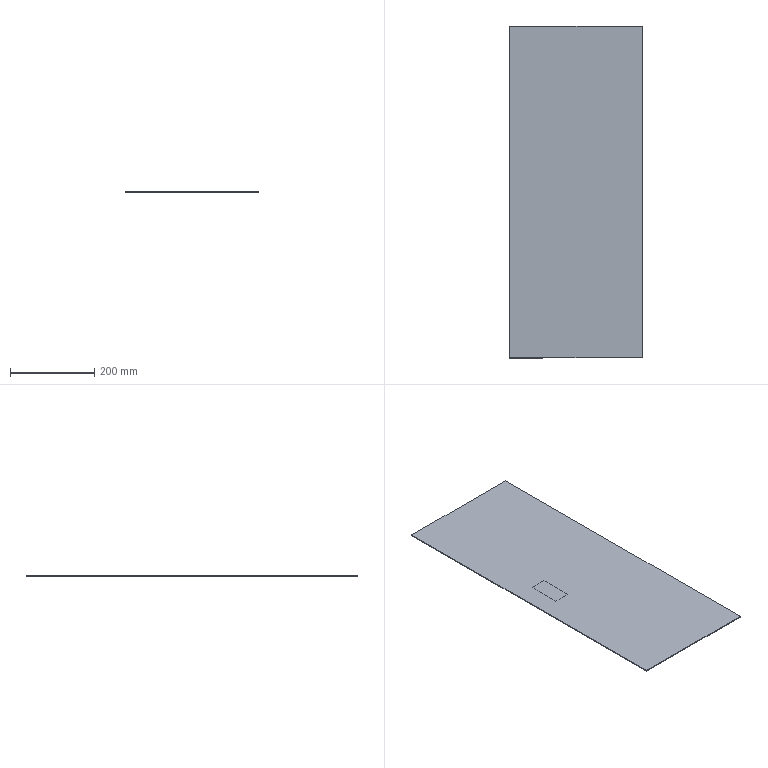Component | SolidWorks | 30-01A-1_ElectricalControlBox-1_DistributionBoxDoor-1 | 1 solid | 11 faces | box 315 x 788 x 2 mm | volume 493240 mm3 | plane 11
build123d program:
from build123d import *

# Parameters (mm, degrees)
SKETCH1_W          = 315
SKETCH1_H          = 788
EXTRUDE1_DEPTH     = 2
SKETCH4_W          = 40
SKETCH4_H          = 80
CUT_EXTRUDE3_DEPTH = 1


with BuildPart() as part:
    # Sketch1 → Extrude1 (new body)
    with BuildSketch(Plane.XY):
        Rectangle(SKETCH1_W, SKETCH1_H)
    extrude(amount=EXTRUDE1_DEPTH)

    # Sketch4 → Cut-Extrude3 (cut)
    with BuildSketch(Plane.XY.offset(2)):
        with Locations((87.5, 0)):
            Rectangle(SKETCH4_W, SKETCH4_H)
    extrude(amount=-CUT_EXTRUDE3_DEPTH, mode=Mode.SUBTRACT)


solid = part.part

# Placed as in the assembly
solid = solid.moved(Location((84.07, -52.845, -1088), (-180, 0, 180)))
STEP:
#1=CARTESIAN_POINT('',(9.511,13.431,-42.835));
#2=VERTEX_POINT('',#1);
#3=CARTESIAN_POINT('',(9.511,-17.592,-42.835));
#4=VERTEX_POINT('',#3);
#5=CARTESIAN_POINT('',(9.511,13.431,-42.835));
#6=DIRECTION('',(0.,-1.,-0.));
#7=VECTOR('',#6,39.37);
#8=LINE('',#5,#7);
#9=EDGE_CURVE('',#2,#4,#8,.T.);
#10=ORIENTED_EDGE('',*,*,#9,.T.);
#11=CARTESIAN_POINT('',(9.511,-17.592,-42.913));
#12=VERTEX_POINT('',#11);
#13=CARTESIAN_POINT('',(9.511,-17.592,-42.913));
#14=DIRECTION('',(0.,-0.,1.));
#15=VECTOR('',#14,39.37);
#16=LINE('',#13,#15);
#17=EDGE_CURVE('',#12,#4,#16,.T.);
#18=ORIENTED_EDGE('',*,*,#17,.F.);
#19=CARTESIAN_POINT('',(9.511,13.431,-42.913));
#20=VERTEX_POINT('',#19);
#21=CARTESIAN_POINT('',(9.511,13.431,-42.913));
#22=DIRECTION('',(0.,-1.,-0.));
#23=VECTOR('',#22,39.37);
#24=LINE('',#21,#23);
#25=EDGE_CURVE('',#20,#12,#24,.T.);
#26=ORIENTED_EDGE('',*,*,#25,.F.);
#27=CARTESIAN_POINT('',(9.511,13.431,-42.913));
#28=DIRECTION('',(0.,-0.,1.));
#29=VECTOR('',#28,39.37);
#30=LINE('',#27,#29);
#31=EDGE_CURVE('',#20,#2,#30,.T.);
#32=ORIENTED_EDGE('',*,*,#31,.T.);
#33=EDGE_LOOP('',(#10,#18,#26,#32));
#34=FACE_OUTER_BOUND('',#33,.T.);
#35=CARTESIAN_POINT('',(9.511,13.431,-42.913));
#36=DIRECTION('',(-1.,-0.,0.));
#37=DIRECTION('',(0.,-0.,1.));
#38=AXIS2_PLACEMENT_3D('',#35,#36,#37);
#39=PLANE('',#38);
#40=ADVANCED_FACE('',(#34),#39,.F.);
#41=CARTESIAN_POINT('',(-2.891,-17.592,-42.835));
#42=VERTEX_POINT('',#41);
#43=CARTESIAN_POINT('',(9.511,-17.592,-42.835));
#44=DIRECTION('',(-1.,-0.,0.));
#45=VECTOR('',#44,39.37);
#46=LINE('',#43,#45);
#47=EDGE_CURVE('',#4,#42,#46,.T.);
#48=ORIENTED_EDGE('',*,*,#47,.T.);
#49=CARTESIAN_POINT('',(-2.891,-17.592,-42.913));
#50=VERTEX_POINT('',#49);
#51=CARTESIAN_POINT('',(-2.891,-17.592,-42.913));
#52=DIRECTION('',(0.,-0.,1.));
#53=VECTOR('',#52,39.37);
#54=LINE('',#51,#53);
#55=EDGE_CURVE('',#50,#42,#54,.T.);
#56=ORIENTED_EDGE('',*,*,#55,.F.);
#57=CARTESIAN_POINT('',(9.511,-17.592,-42.913));
#58=DIRECTION('',(-1.,-0.,0.));
#59=VECTOR('',#58,39.37);
#60=LINE('',#57,#59);
#61=EDGE_CURVE('',#12,#50,#60,.T.);
#62=ORIENTED_EDGE('',*,*,#61,.F.);
#63=ORIENTED_EDGE('',*,*,#17,.T.);
#64=EDGE_LOOP('',(#48,#56,#62,#63));
#65=FACE_OUTER_BOUND('',#64,.T.);
#66=CARTESIAN_POINT('',(9.511,-17.592,-42.913));
#67=DIRECTION('',(-0.,1.,0.));
#68=DIRECTION('',(-0.,0.,-1.));
#69=AXIS2_PLACEMENT_3D('',#66,#67,#68);
#70=PLANE('',#69);
#71=ADVANCED_FACE('',(#65),#70,.F.);
#72=CARTESIAN_POINT('',(-2.891,13.431,-42.835));
#73=VERTEX_POINT('',#72);
#74=CARTESIAN_POINT('',(-2.891,13.431,-42.835));
#75=DIRECTION('',(-0.,1.,0.));
#76=VECTOR('',#75,39.37);
#77=LINE('',#74,#76);
#78=EDGE_CURVE('',#42,#73,#77,.T.);
#79=ORIENTED_EDGE('',*,*,#78,.T.);
#80=CARTESIAN_POINT('',(-2.891,13.431,-42.913));
#81=VERTEX_POINT('',#80);
#82=CARTESIAN_POINT('',(-2.891,13.431,-42.913));
#83=DIRECTION('',(0.,-0.,1.));
#84=VECTOR('',#83,39.37);
#85=LINE('',#82,#84);
#86=EDGE_CURVE('',#81,#73,#85,.T.);
#87=ORIENTED_EDGE('',*,*,#86,.F.);
#88=CARTESIAN_POINT('',(-2.891,13.431,-42.913));
#89=DIRECTION('',(-0.,1.,0.));
#90=VECTOR('',#89,39.37);
#91=LINE('',#88,#90);
#92=EDGE_CURVE('',#50,#81,#91,.T.);
#93=ORIENTED_EDGE('',*,*,#92,.F.);
#94=ORIENTED_EDGE('',*,*,#55,.T.);
#95=EDGE_LOOP('',(#79,#87,#93,#94));
#96=FACE_OUTER_BOUND('',#95,.T.);
#97=CARTESIAN_POINT('',(-2.891,13.431,-42.913));
#98=DIRECTION('',(1.,0.,-0.));
#99=DIRECTION('',(-0.,0.,-1.));
#100=AXIS2_PLACEMENT_3D('',#97,#98,#99);
#101=PLANE('',#100);
#102=ADVANCED_FACE('',(#96),#101,.F.);
#103=CARTESIAN_POINT('',(9.511,13.431,-42.835));
#104=DIRECTION('',(1.,0.,-0.));
#105=VECTOR('',#104,39.37);
#106=LINE('',#103,#105);
#107=EDGE_CURVE('',#73,#2,#106,.T.);
#108=ORIENTED_EDGE('',*,*,#107,.T.);
#109=ORIENTED_EDGE('',*,*,#31,.F.);
#110=CARTESIAN_POINT('',(9.511,13.431,-42.913));
#111=DIRECTION('',(1.,0.,-0.));
#112=VECTOR('',#111,39.37);
#113=LINE('',#110,#112);
#114=EDGE_CURVE('',#81,#20,#113,.T.);
#115=ORIENTED_EDGE('',*,*,#114,.F.);
#116=ORIENTED_EDGE('',*,*,#86,.T.);
#117=EDGE_LOOP('',(#108,#109,#115,#116));
#118=FACE_OUTER_BOUND('',#117,.T.);
#119=CARTESIAN_POINT('',(9.511,13.431,-42.913));
#120=DIRECTION('',(0.,-1.,-0.));
#121=DIRECTION('',(0.,-0.,1.));
#122=AXIS2_PLACEMENT_3D('',#119,#120,#121);
#123=PLANE('',#122);
#124=ADVANCED_FACE('',(#118),#123,.F.);
#125=CARTESIAN_POINT('',(0.6524,-0.5057,-42.913));
#126=VERTEX_POINT('',#125);
#127=CARTESIAN_POINT('',(0.6524,-3.655,-42.913));
#128=VERTEX_POINT('',#127);
#129=CARTESIAN_POINT('',(0.6524,-0.5057,-42.913));
#130=DIRECTION('',(0.,-1.,-0.));
#131=VECTOR('',#130,39.37);
#132=LINE('',#129,#131);
#133=EDGE_CURVE('',#126,#128,#132,.T.);
#134=ORIENTED_EDGE('',*,*,#133,.F.);
#135=CARTESIAN_POINT('',(-0.9224,-0.5057,-42.913));
#136=VERTEX_POINT('',#135);
#137=CARTESIAN_POINT('',(0.6524,-0.5057,-42.913));
#138=DIRECTION('',(1.,0.,-0.));
#139=VECTOR('',#138,39.37);
#140=LINE('',#137,#139);
#141=EDGE_CURVE('',#136,#126,#140,.T.);
#142=ORIENTED_EDGE('',*,*,#141,.F.);
#143=CARTESIAN_POINT('',(-0.9224,-3.655,-42.913));
#144=VERTEX_POINT('',#143);
#145=CARTESIAN_POINT('',(-0.9224,-0.5057,-42.913));
#146=DIRECTION('',(-0.,1.,0.));
#147=VECTOR('',#146,39.37);
#148=LINE('',#145,#147);
#149=EDGE_CURVE('',#144,#136,#148,.T.);
#150=ORIENTED_EDGE('',*,*,#149,.F.);
#151=CARTESIAN_POINT('',(0.6524,-3.655,-42.913));
#152=DIRECTION('',(-1.,-0.,0.));
#153=VECTOR('',#152,39.37);
#154=LINE('',#151,#153);
#155=EDGE_CURVE('',#128,#144,#154,.T.);
#156=ORIENTED_EDGE('',*,*,#155,.F.);
#157=EDGE_LOOP('',(#134,#142,#150,#156));
#158=FACE_BOUND('',#157,.T.);
#159=ORIENTED_EDGE('',*,*,#25,.T.);
#160=ORIENTED_EDGE('',*,*,#61,.T.);
#161=ORIENTED_EDGE('',*,*,#92,.T.);
#162=ORIENTED_EDGE('',*,*,#114,.T.);
#163=EDGE_LOOP('',(#159,#160,#161,#162));
#164=FACE_OUTER_BOUND('',#163,.T.);
#165=CARTESIAN_POINT('',(9.511,-17.592,-42.913));
#166=DIRECTION('',(-0.,0.,-1.));
#167=DIRECTION('',(-1.,-0.,0.));
#168=AXIS2_PLACEMENT_3D('',#165,#166,#167);
#169=PLANE('',#168);
#170=ADVANCED_FACE('',(#158,#164),#169,.T.);
#171=ORIENTED_EDGE('',*,*,#9,.F.);
#172=ORIENTED_EDGE('',*,*,#107,.F.);
#173=ORIENTED_EDGE('',*,*,#78,.F.);
#174=ORIENTED_EDGE('',*,*,#47,.F.);
#175=EDGE_LOOP('',(#171,#172,#173,#174));
#176=FACE_OUTER_BOUND('',#175,.T.);
#177=CARTESIAN_POINT('',(9.511,-17.592,-42.835));
#178=DIRECTION('',(-0.,0.,-1.));
#179=DIRECTION('',(-1.,-0.,0.));
#180=AXIS2_PLACEMENT_3D('',#177,#178,#179);
#181=PLANE('',#180);
#182=ADVANCED_FACE('',(#176),#181,.F.);
#183=ORIENTED_EDGE('',*,*,#133,.T.);
#184=CARTESIAN_POINT('',(0.6524,-3.655,-42.874));
#185=VERTEX_POINT('',#184);
#186=CARTESIAN_POINT('',(0.6524,-3.655,-42.874));
#187=DIRECTION('',(-0.,0.,-1.));
#188=VECTOR('',#187,39.37);
#189=LINE('',#186,#188);
#190=EDGE_CURVE('',#185,#128,#189,.T.);
#191=ORIENTED_EDGE('',*,*,#190,.F.);
#192=CARTESIAN_POINT('',(0.6524,-0.5057,-42.874));
#193=VERTEX_POINT('',#192);
#194=CARTESIAN_POINT('',(0.6524,-0.5057,-42.874));
#195=DIRECTION('',(0.,-1.,-0.));
#196=VECTOR('',#195,39.37);
#197=LINE('',#194,#196);
#198=EDGE_CURVE('',#193,#185,#197,.T.);
#199=ORIENTED_EDGE('',*,*,#198,.F.);
#200=CARTESIAN_POINT('',(0.6524,-0.5057,-42.874));
#201=DIRECTION('',(-0.,0.,-1.));
#202=VECTOR('',#201,39.37);
#203=LINE('',#200,#202);
#204=EDGE_CURVE('',#193,#126,#203,.T.);
#205=ORIENTED_EDGE('',*,*,#204,.T.);
#206=EDGE_LOOP('',(#183,#191,#199,#205));
#207=FACE_OUTER_BOUND('',#206,.T.);
#208=CARTESIAN_POINT('',(0.6524,-0.5057,-42.874));
#209=DIRECTION('',(1.,0.,-0.));
#210=DIRECTION('',(0.,-1.,-0.));
#211=AXIS2_PLACEMENT_3D('',#208,#209,#210);
#212=PLANE('',#211);
#213=ADVANCED_FACE('',(#207),#212,.F.);
#214=ORIENTED_EDGE('',*,*,#141,.T.);
#215=ORIENTED_EDGE('',*,*,#204,.F.);
#216=CARTESIAN_POINT('',(-0.9224,-0.5057,-42.874));
#217=VERTEX_POINT('',#216);
#218=CARTESIAN_POINT('',(0.6524,-0.5057,-42.874));
#219=DIRECTION('',(1.,0.,-0.));
#220=VECTOR('',#219,39.37);
#221=LINE('',#218,#220);
#222=EDGE_CURVE('',#217,#193,#221,.T.);
#223=ORIENTED_EDGE('',*,*,#222,.F.);
#224=CARTESIAN_POINT('',(-0.9224,-0.5057,-42.874));
#225=DIRECTION('',(-0.,0.,-1.));
#226=VECTOR('',#225,39.37);
#227=LINE('',#224,#226);
#228=EDGE_CURVE('',#217,#136,#227,.T.);
#229=ORIENTED_EDGE('',*,*,#228,.T.);
#230=EDGE_LOOP('',(#214,#215,#223,#229));
#231=FACE_OUTER_BOUND('',#230,.T.);
#232=CARTESIAN_POINT('',(0.6524,-0.5057,-42.874));
#233=DIRECTION('',(-0.,1.,0.));
#234=DIRECTION('',(1.,0.,-0.));
#235=AXIS2_PLACEMENT_3D('',#232,#233,#234);
#236=PLANE('',#235);
#237=ADVANCED_FACE('',(#231),#236,.F.);
#238=ORIENTED_EDGE('',*,*,#149,.T.);
#239=ORIENTED_EDGE('',*,*,#228,.F.);
#240=CARTESIAN_POINT('',(-0.9224,-3.655,-42.874));
#241=VERTEX_POINT('',#240);
#242=CARTESIAN_POINT('',(-0.9224,-0.5057,-42.874));
#243=DIRECTION('',(-0.,1.,0.));
#244=VECTOR('',#243,39.37);
#245=LINE('',#242,#244);
#246=EDGE_CURVE('',#241,#217,#245,.T.);
#247=ORIENTED_EDGE('',*,*,#246,.F.);
#248=CARTESIAN_POINT('',(-0.9224,-3.655,-42.874));
#249=DIRECTION('',(-0.,0.,-1.));
#250=VECTOR('',#249,39.37);
#251=LINE('',#248,#250);
#252=EDGE_CURVE('',#241,#144,#251,.T.);
#253=ORIENTED_EDGE('',*,*,#252,.T.);
#254=EDGE_LOOP('',(#238,#239,#247,#253));
#255=FACE_OUTER_BOUND('',#254,.T.);
#256=CARTESIAN_POINT('',(-0.9224,-0.5057,-42.874));
#257=DIRECTION('',(-1.,-0.,0.));
#258=DIRECTION('',(-0.,1.,0.));
#259=AXIS2_PLACEMENT_3D('',#256,#257,#258);
#260=PLANE('',#259);
#261=ADVANCED_FACE('',(#255),#260,.F.);
#262=ORIENTED_EDGE('',*,*,#155,.T.);
#263=ORIENTED_EDGE('',*,*,#252,.F.);
#264=CARTESIAN_POINT('',(0.6524,-3.655,-42.874));
#265=DIRECTION('',(-1.,-0.,0.));
#266=VECTOR('',#265,39.37);
#267=LINE('',#264,#266);
#268=EDGE_CURVE('',#185,#241,#267,.T.);
#269=ORIENTED_EDGE('',*,*,#268,.F.);
#270=ORIENTED_EDGE('',*,*,#190,.T.);
#271=EDGE_LOOP('',(#262,#263,#269,#270));
#272=FACE_OUTER_BOUND('',#271,.T.);
#273=CARTESIAN_POINT('',(0.6524,-3.655,-42.874));
#274=DIRECTION('',(0.,-1.,-0.));
#275=DIRECTION('',(0.,-0.,1.));
#276=AXIS2_PLACEMENT_3D('',#273,#274,#275);
#277=PLANE('',#276);
#278=ADVANCED_FACE('',(#272),#277,.F.);
#279=ORIENTED_EDGE('',*,*,#198,.T.);
#280=ORIENTED_EDGE('',*,*,#268,.T.);
#281=ORIENTED_EDGE('',*,*,#246,.T.);
#282=ORIENTED_EDGE('',*,*,#222,.T.);
#283=EDGE_LOOP('',(#279,#280,#281,#282));
#284=FACE_OUTER_BOUND('',#283,.T.);
#285=CARTESIAN_POINT('',(0.6524,-3.655,-42.874));
#286=DIRECTION('',(-0.,0.,-1.));
#287=DIRECTION('',(-1.,-0.,0.));
#288=AXIS2_PLACEMENT_3D('',#285,#286,#287);
#289=PLANE('',#288);
#290=ADVANCED_FACE('',(#284),#289,.T.);
#291=CLOSED_SHELL('',(#40,#71,#102,#124,#170,#182,#213,#237,#261,#278,#290));
#292=MANIFOLD_SOLID_BREP('',#291);
#293=CARTESIAN_POINT('',(0.,0.,0.));
#294=DIRECTION('',(0.,0.,1.));
#295=DIRECTION('',(1.,0.,0.));
#296=AXIS2_PLACEMENT_3D('',#293,#294,#295);
#297=(LENGTH_UNIT()NAMED_UNIT(*)SI_UNIT($,.METRE.));
#298=LENGTH_MEASURE_WITH_UNIT(LENGTH_MEASURE(0.0254),#297);
#299=DIMENSIONAL_EXPONENTS(1.,0.,0.,0.,0.,0.,0.);
#300=(CONVERSION_BASED_UNIT('',#298)LENGTH_UNIT()NAMED_UNIT(#299));
#301=UNCERTAINTY_MEASURE_WITH_UNIT(LENGTH_MEASURE(0.00001),#300,'','');
#302=(NAMED_UNIT(*)PLANE_ANGLE_UNIT()SI_UNIT($,.RADIAN.));
#303=(NAMED_UNIT(*)SI_UNIT($,.STERADIAN.)SOLID_ANGLE_UNIT());
#304=(GEOMETRIC_REPRESENTATION_CONTEXT(3)GLOBAL_UNCERTAINTY_ASSIGNED_CONTEXT((#301))GLOBAL_UNIT_ASSIGNED_CONTEXT((#300,#302,#303))REPRESENTATION_CONTEXT('',''));
#305=ADVANCED_BREP_SHAPE_REPRESENTATION('',(#292,#296),#304);
#306=COLOUR_RGB('',0.7922,0.8196,0.9333);
#307=FILL_AREA_STYLE_COLOUR('',#306);
#308=FILL_AREA_STYLE('',(#307));
#309=SURFACE_STYLE_FILL_AREA(#308);
#310=SURFACE_SIDE_STYLE('',(#309));
#311=SURFACE_STYLE_USAGE(.BOTH.,#310);
#312=PRESENTATION_STYLE_ASSIGNMENT((#311));
#313=STYLED_ITEM('',(#312),#292);
#314=PRESENTATION_LAYER_ASSIGNMENT('','',(#313));
#315=(LENGTH_UNIT()NAMED_UNIT(*)SI_UNIT($,.METRE.));
#316=LENGTH_MEASURE_WITH_UNIT(LENGTH_MEASURE(0.0254),#315);
#317=DIMENSIONAL_EXPONENTS(1.,0.,0.,0.,0.,0.,0.);
#318=(CONVERSION_BASED_UNIT('',#316)LENGTH_UNIT()NAMED_UNIT(#317));
#319=UNCERTAINTY_MEASURE_WITH_UNIT(LENGTH_MEASURE(0.00001),#318,'','');
#320=(NAMED_UNIT(*)PLANE_ANGLE_UNIT()SI_UNIT($,.RADIAN.));
#321=(NAMED_UNIT(*)SI_UNIT($,.STERADIAN.)SOLID_ANGLE_UNIT());
#322=(GEOMETRIC_REPRESENTATION_CONTEXT(3)GLOBAL_UNCERTAINTY_ASSIGNED_CONTEXT((#319))GLOBAL_UNIT_ASSIGNED_CONTEXT((#318,#320,#321))REPRESENTATION_CONTEXT('',''));
#323=MECHANICAL_DESIGN_GEOMETRIC_PRESENTATION_REPRESENTATION('',(#313),#322);